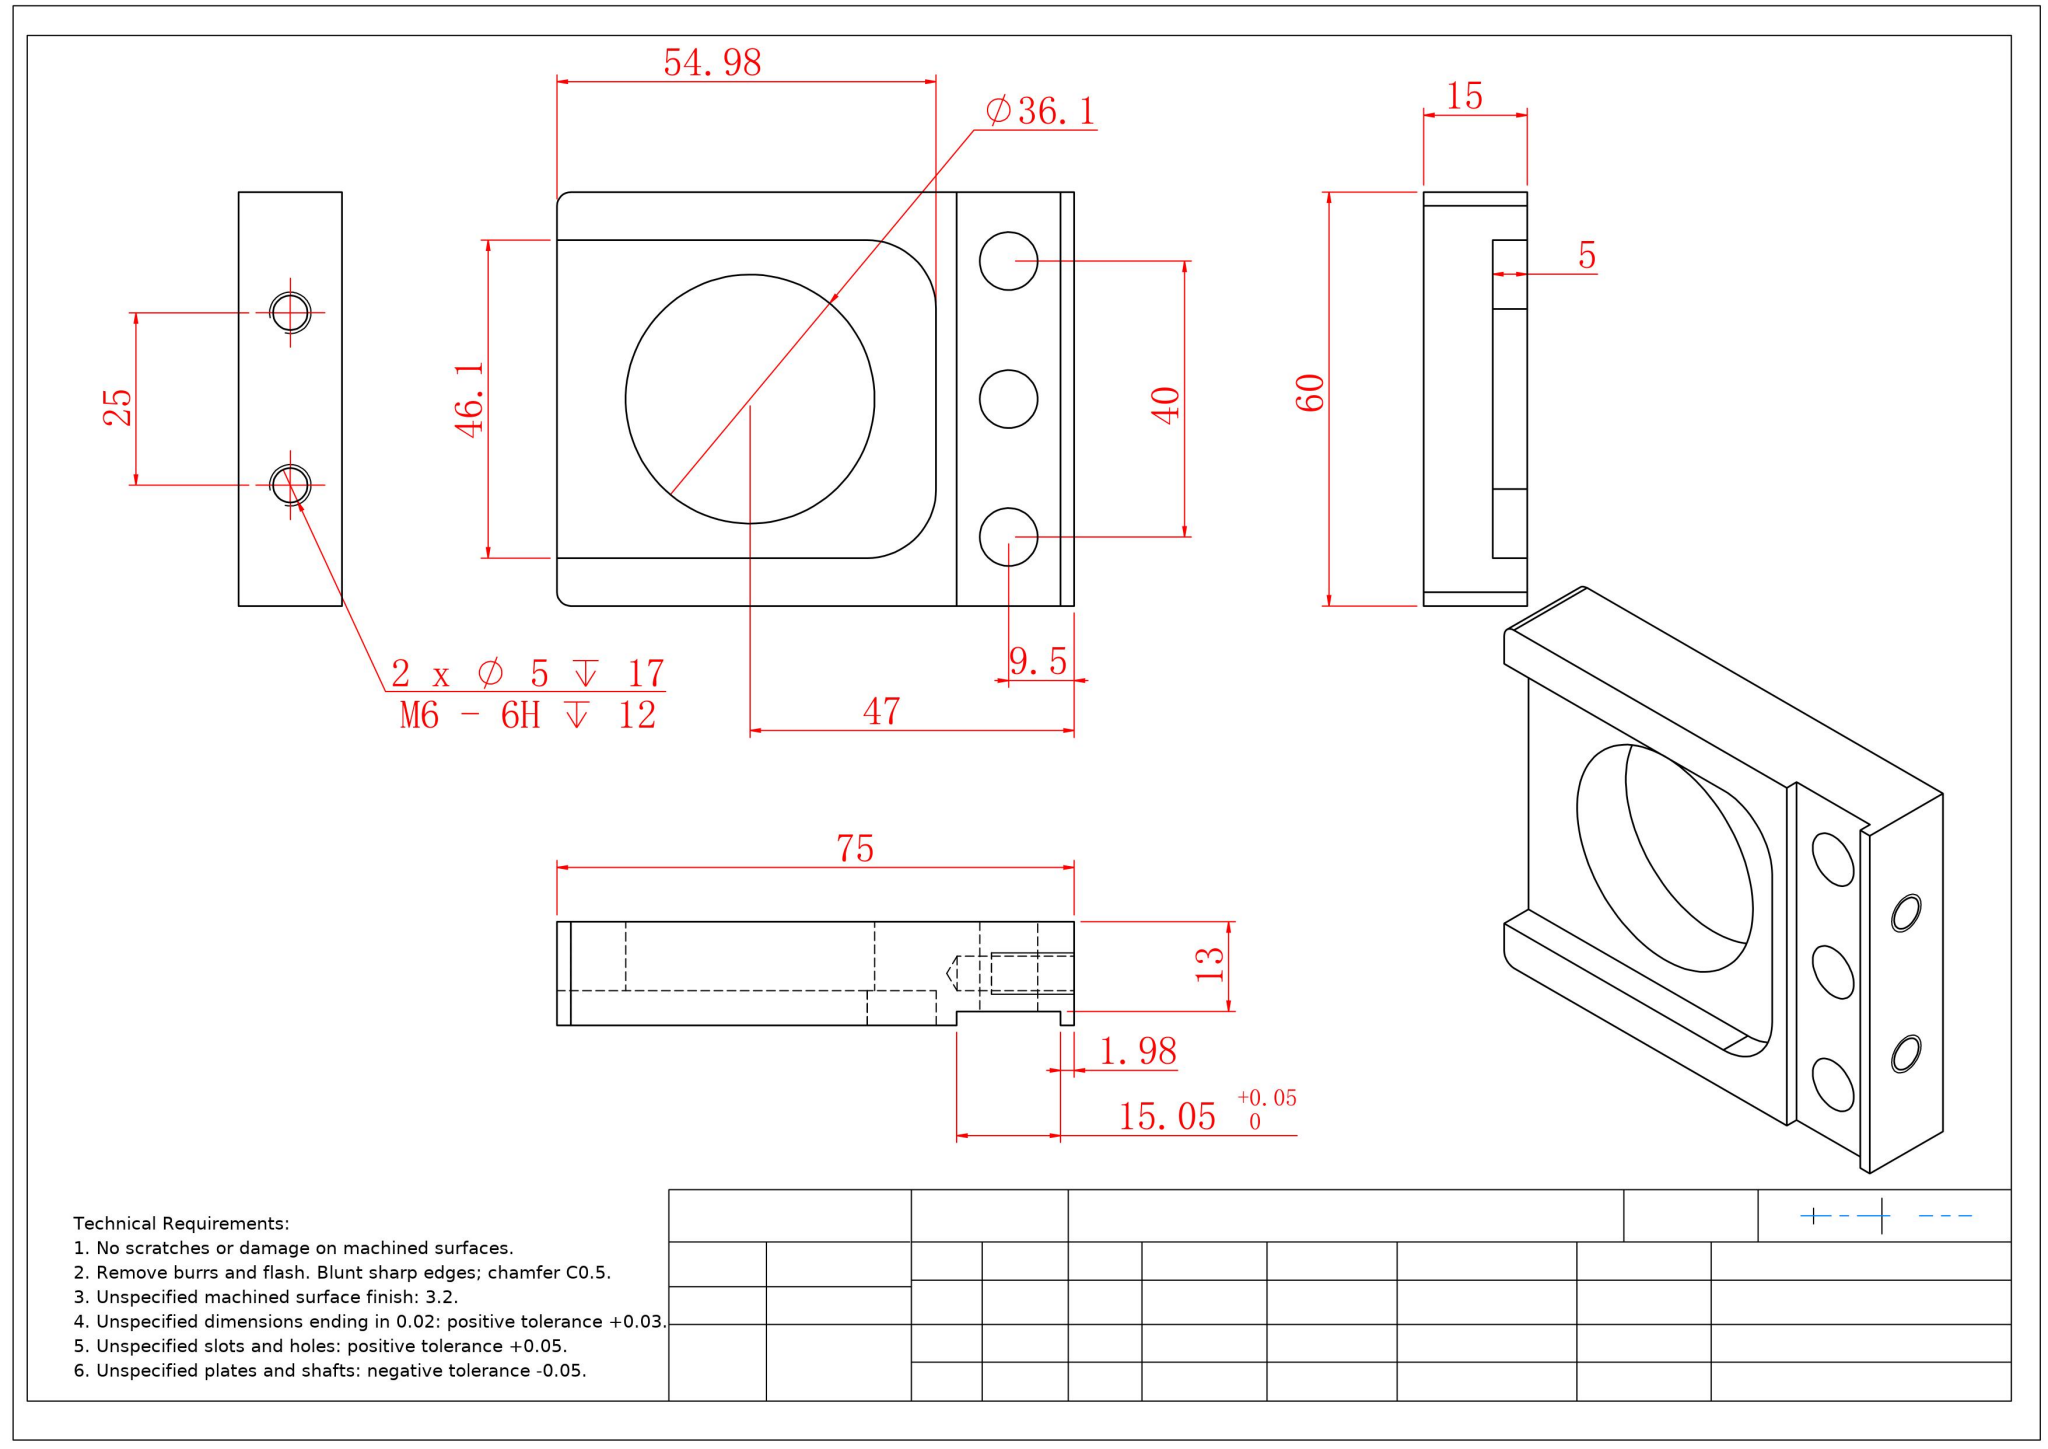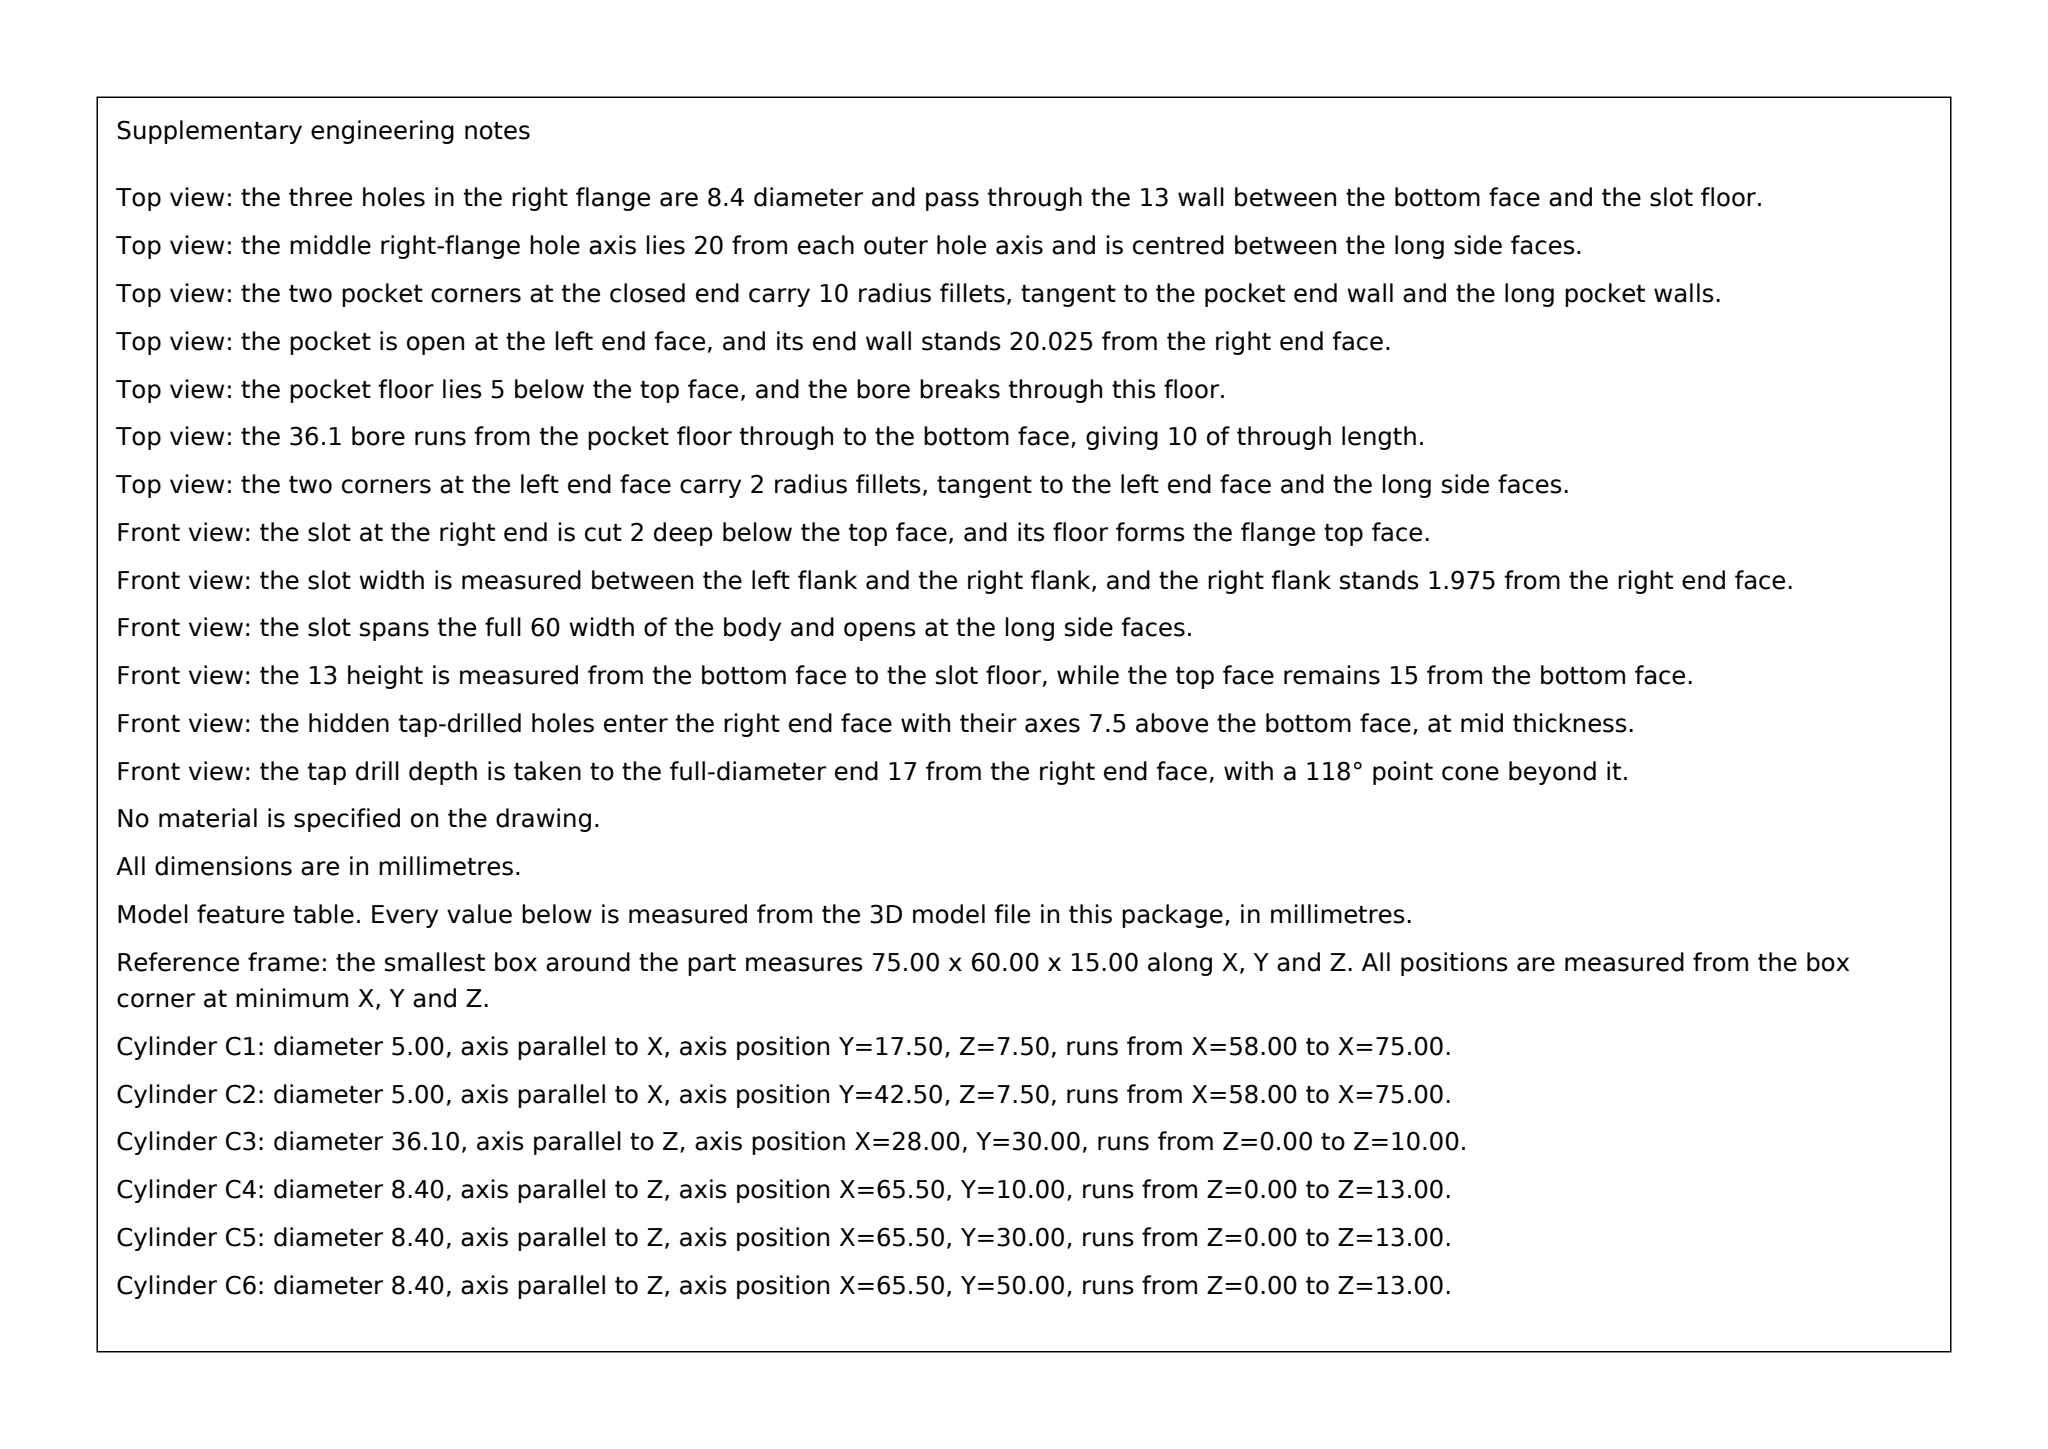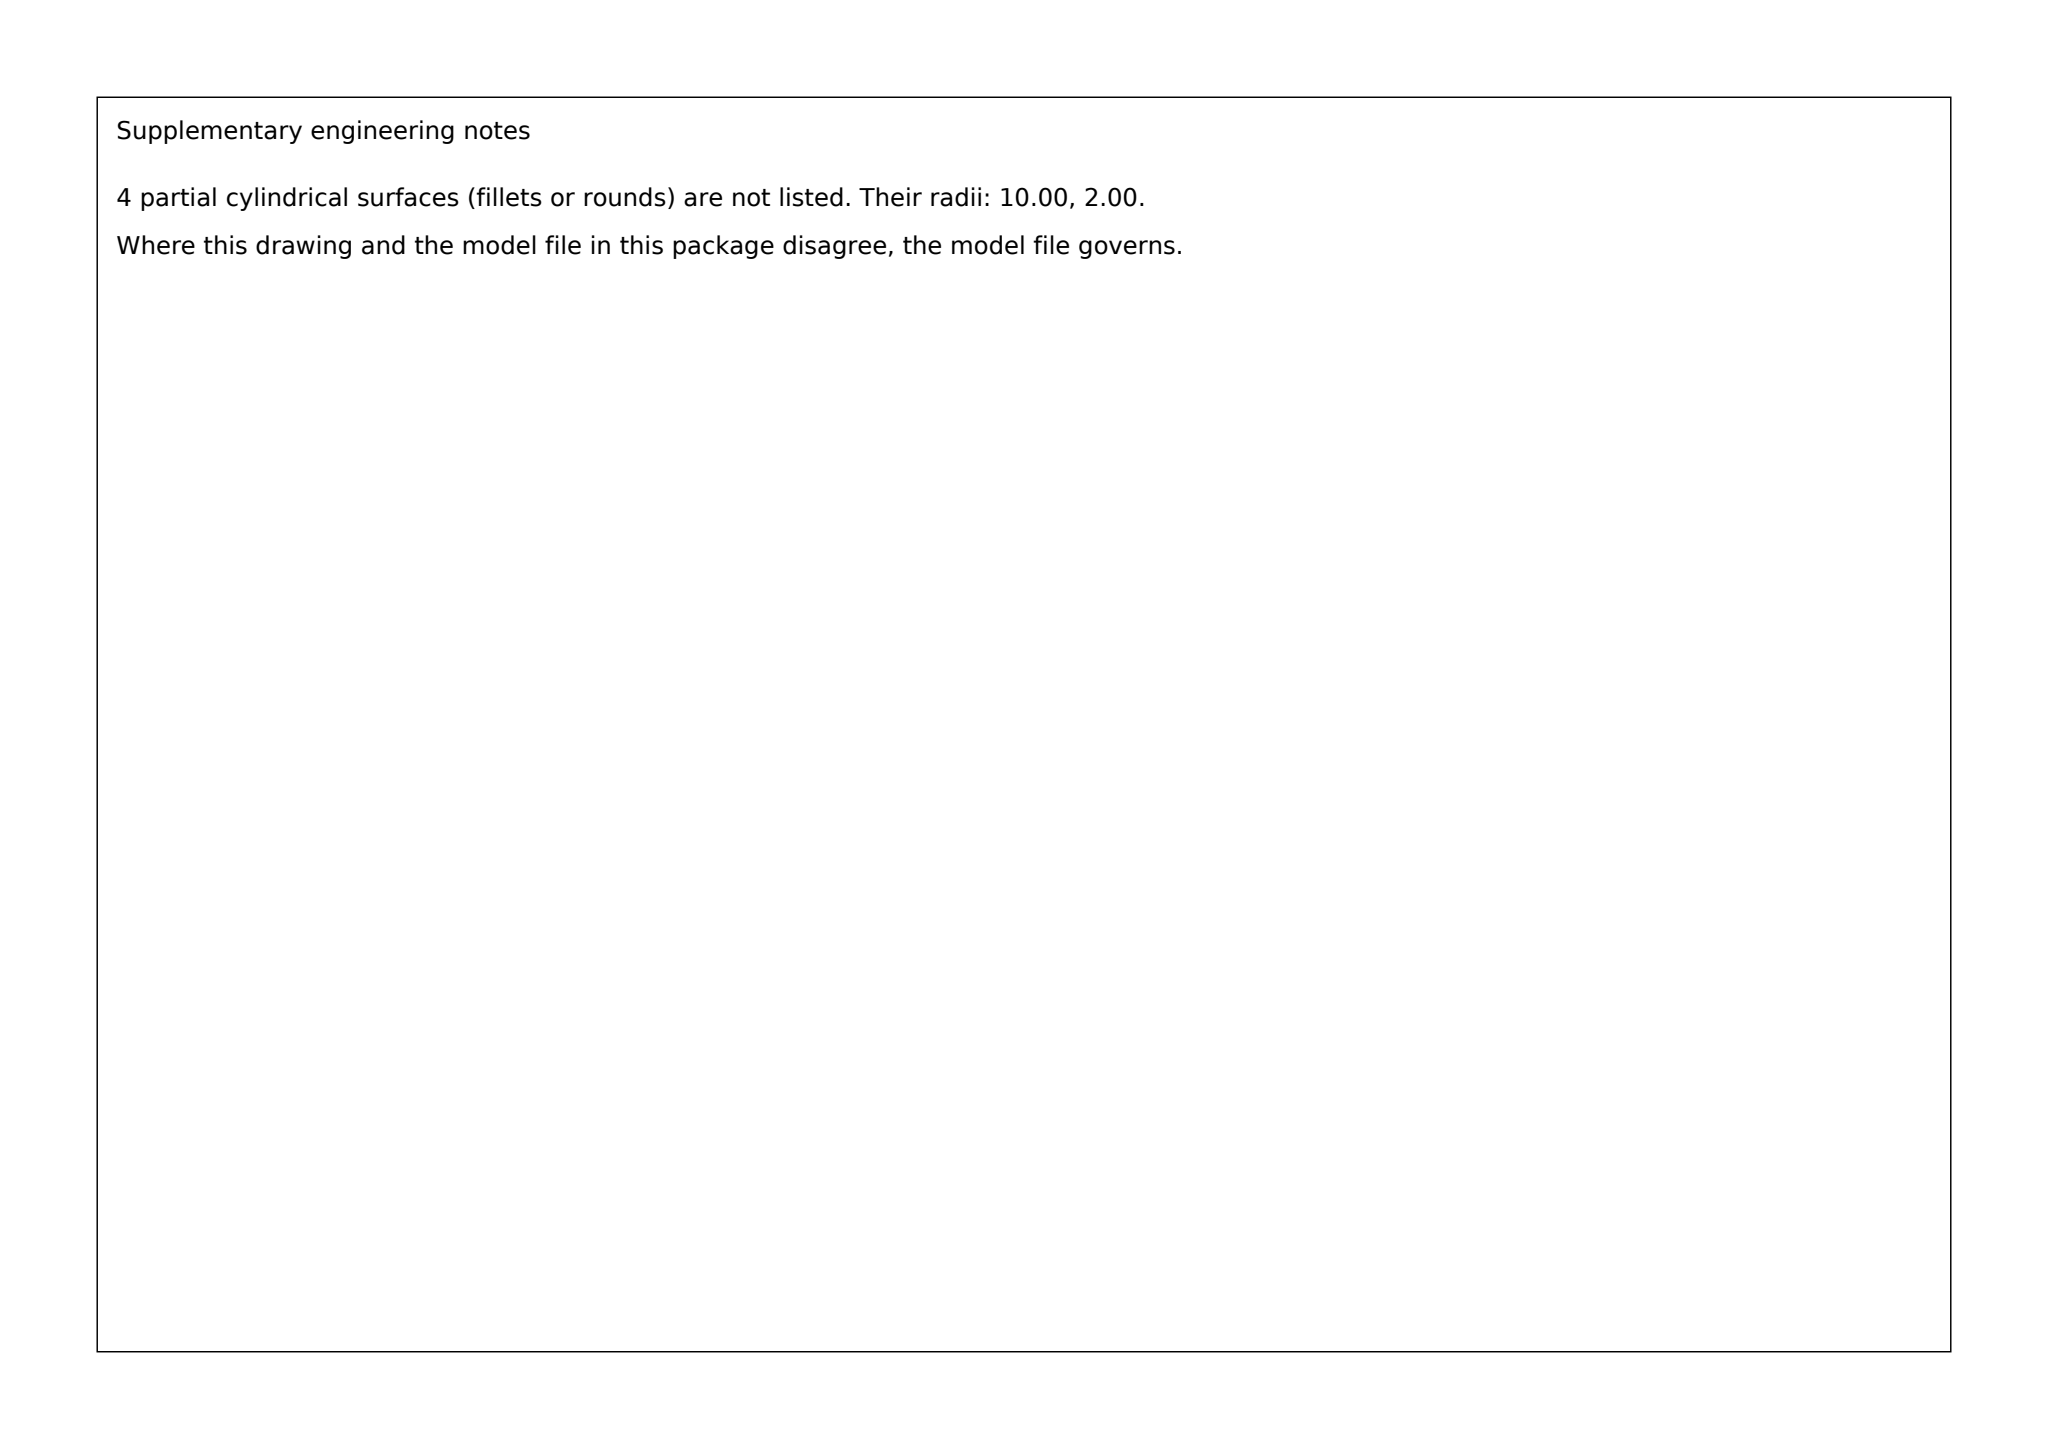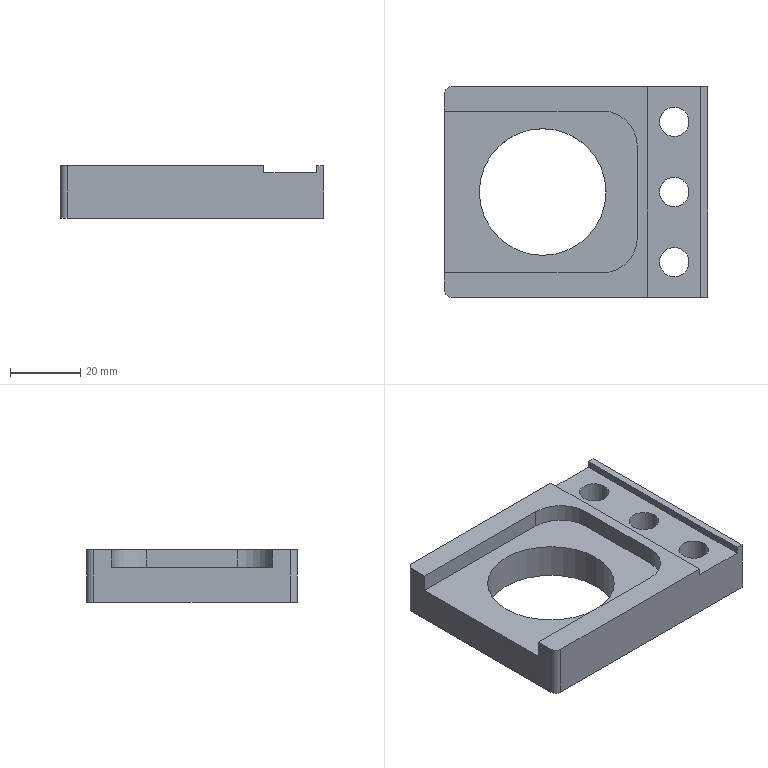Part | SolidWorks | mm | 1 solid | 34 faces | box 75 x 60 x 15 mm | volume 40127 mm3 | cylinder 16 | plane 14 | cone 4 | commonest cylinder face diameters 8.4 x6 5 x4 36.1 x2 20 x2 4 x2